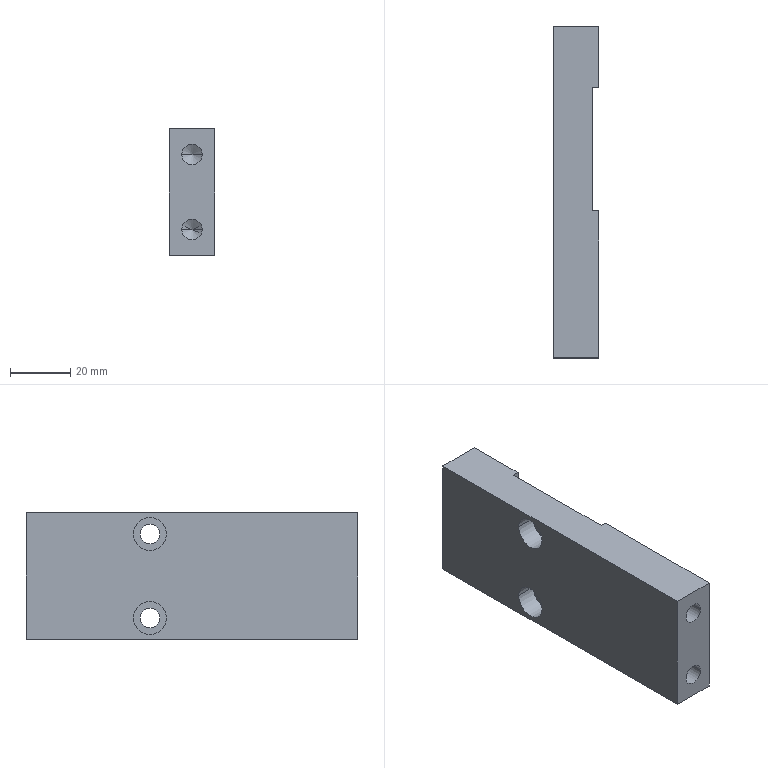Component | SolidWorks | CylinderBracket2-1 | 1 solid | 36 faces | box 15 x 110.5 x 42 mm | volume 62147 mm3 | cylinder 16 | plane 12 | cone 8 | commonest cylinder face diameters 3.3 x4 11 x4 6.6 x4 6.8 x4
build123d program:
from build123d import *

# Parameters (mm, degrees)
SKETCH2_W                                       = 15
SKETCH2_H                                       = 42
BOSS_EXTRUDE1_DEPTH                             = 138.5
M8_TAPPED_HOLE1_D                               = 6.8
M8_TAPPED_HOLE1_DEPTH                           = 25
M8_TAPPED_HOLE1_TIP                             = 2.043
SKETCH7_W                                       = 2
SKETCH7_H                                       = 41.1
CUT_EXTRUDE1_DEPTH                              = 42
M6_HEX_SOCKET_HEAD_CAP_SCREW_CBORE1_D           = 6.6
M6_HEX_SOCKET_HEAD_CAP_SCREW_CBORE1_CBORE_D     = 11
M6_HEX_SOCKET_HEAD_CAP_SCREW_CBORE1_CBORE_DEPTH = 6.8
SKETCH10_W                                      = 15
SKETCH10_H                                      = 28
CUT_EXTRUDE2_DEPTH                              = 53
M4_TAPPED_HOLE1_D                               = 3.3
M4_TAPPED_HOLE1_DEPTH                           = 25
M4_TAPPED_HOLE1_TIP                             = 0.9914


with BuildPart() as part:
    # Sketch2 → Boss-Extrude1 (new body)
    with BuildSketch(Plane.XY):
        with Locations((-3.66, -1.392)):
            Rectangle(SKETCH2_W, SKETCH2_H)
    extrude(amount=BOSS_EXTRUDE1_DEPTH)

    # M8 Tapped Hole1
    with Locations(Plane.XY.offset(138.5)):
        with Locations((-3.66, 11.108), (-3.66, -13.892)):
            Hole(M8_TAPPED_HOLE1_D / 2, depth=M8_TAPPED_HOLE1_DEPTH)
            with Locations((0, 0, -(M8_TAPPED_HOLE1_DEPTH + M8_TAPPED_HOLE1_TIP / 2))):  # 118° drill point
                Cone(0, M8_TAPPED_HOLE1_D / 2, M8_TAPPED_HOLE1_TIP, mode=Mode.SUBTRACT)

    # Sketch7 → Cut-Extrude1 (cut)
    with BuildSketch(Plane.XZ.offset(22.392)):
        with Locations((2.84, 69)):
            Rectangle(SKETCH7_W, SKETCH7_H)
    extrude(amount=-CUT_EXTRUDE1_DEPTH, mode=Mode.SUBTRACT)

    # M6 Hex Socket Head Cap Screw CBORE1 (through all)
    with Locations(Plane.ZY.offset(11.16)):
        with Locations((69.25, 12.608), (69.25, -15.392)):
            CounterBoreHole(M6_HEX_SOCKET_HEAD_CAP_SCREW_CBORE1_D / 2, M6_HEX_SOCKET_HEAD_CAP_SCREW_CBORE1_CBORE_D / 2, M6_HEX_SOCKET_HEAD_CAP_SCREW_CBORE1_CBORE_DEPTH)

    # Sketch10 → Cut-Extrude2 (cut)
    with BuildSketch(Plane.XZ.offset(22.392)):
        with Locations((-3.66, 14)):
            Rectangle(SKETCH10_W, SKETCH10_H)
    extrude(amount=-CUT_EXTRUDE2_DEPTH, mode=Mode.SUBTRACT)

    # M4 Tapped Hole1
    with Locations(Plane(origin=(0, 0, 28), x_dir=(-1, 0, 0), z_dir=(0, 0, -1))):
        with Locations((3.66, -18.392), (3.66, 15.608)):
            Hole(M4_TAPPED_HOLE1_D / 2, depth=M4_TAPPED_HOLE1_DEPTH)
            with Locations((0, 0, -(M4_TAPPED_HOLE1_DEPTH + M4_TAPPED_HOLE1_TIP / 2))):  # 118° drill point
                Cone(0, M4_TAPPED_HOLE1_D / 2, M4_TAPPED_HOLE1_TIP, mode=Mode.SUBTRACT)


solid = part.part

# Placed as in the assembly
solid = solid.moved(Location((-635.536, -9.151, 375.56), (90, 0, 0)))
STEP:
#1=CARTESIAN_POINT('',(-25.165,-2.447,13.997));
#2=VERTEX_POINT('',#1);
#3=CARTESIAN_POINT('',(-25.165,-2.447,14.127));
#4=VERTEX_POINT('',#3);
#5=CARTESIAN_POINT('',(-25.165,-2.447,14.062));
#6=DIRECTION('',(-0.,1.,-0.));
#7=DIRECTION('',(0.,0.,1.));
#8=AXIS2_PLACEMENT_3D('',#5,#6,#7);
#9=CIRCLE('',#8,0.06496);
#10=EDGE_CURVE('',#2,#4,#9,.T.);
#11=ORIENTED_EDGE('',*,*,#10,.F.);
#12=CARTESIAN_POINT('',(-25.165,-1.463,13.997));
#13=VERTEX_POINT('',#12);
#14=CARTESIAN_POINT('',(-25.165,-1.463,13.997));
#15=DIRECTION('',(-0.,1.,-0.));
#16=VECTOR('',#15,39.37);
#17=LINE('',#14,#16);
#18=EDGE_CURVE('',#2,#13,#17,.T.);
#19=ORIENTED_EDGE('',*,*,#18,.T.);
#20=CARTESIAN_POINT('',(-25.165,-1.463,14.127));
#21=VERTEX_POINT('',#20);
#22=CARTESIAN_POINT('',(-25.165,-1.463,14.062));
#23=DIRECTION('',(-0.,1.,-0.));
#24=DIRECTION('',(0.,0.,1.));
#25=AXIS2_PLACEMENT_3D('',#22,#23,#24);
#26=CIRCLE('',#25,0.06496);
#27=EDGE_CURVE('',#13,#21,#26,.T.);
#28=ORIENTED_EDGE('',*,*,#27,.T.);
#29=CARTESIAN_POINT('',(-25.165,-1.463,14.127));
#30=DIRECTION('',(-0.,1.,-0.));
#31=VECTOR('',#30,39.37);
#32=LINE('',#29,#31);
#33=EDGE_CURVE('',#4,#21,#32,.T.);
#34=ORIENTED_EDGE('',*,*,#33,.F.);
#35=EDGE_LOOP('',(#11,#19,#28,#34));
#36=FACE_OUTER_BOUND('',#35,.T.);
#37=CARTESIAN_POINT('',(-25.165,-1.463,14.062));
#38=DIRECTION('',(-0.,1.,-0.));
#39=DIRECTION('',(0.,0.,1.));
#40=AXIS2_PLACEMENT_3D('',#37,#38,#39);
#41=CYLINDRICAL_SURFACE('',#40,0.06496);
#42=ADVANCED_FACE('',(#36),#41,.F.);
#43=CARTESIAN_POINT('',(-25.165,-2.486,14.062));
#44=VERTEX_POINT('',#43);
#45=CARTESIAN_POINT('',(-25.165,-2.447,14.127));
#46=DIRECTION('',(-0.,0.515,0.8572));
#47=VECTOR('',#46,39.37);
#48=LINE('',#45,#47);
#49=EDGE_CURVE('',#44,#4,#48,.T.);
#50=ORIENTED_EDGE('',*,*,#49,.F.);
#51=CARTESIAN_POINT('',(-25.165,-2.447,13.997));
#52=DIRECTION('',(0.,0.515,-0.8572));
#53=VECTOR('',#52,39.37);
#54=LINE('',#51,#53);
#55=EDGE_CURVE('',#44,#2,#54,.T.);
#56=ORIENTED_EDGE('',*,*,#55,.T.);
#57=ORIENTED_EDGE('',*,*,#10,.T.);
#58=EDGE_LOOP('',(#50,#56,#57));
#59=FACE_OUTER_BOUND('',#58,.T.);
#60=CARTESIAN_POINT('',(-25.165,-2.447,14.062));
#61=DIRECTION('',(-0.,1.,-0.));
#62=DIRECTION('',(0.,0.,1.));
#63=AXIS2_PLACEMENT_3D('',#60,#61,#62);
#64=CONICAL_SURFACE('',#63,0.06496,1.03);
#65=ADVANCED_FACE('',(#59),#64,.F.);
#66=CARTESIAN_POINT('',(-25.165,-2.447,15.335));
#67=VERTEX_POINT('',#66);
#68=CARTESIAN_POINT('',(-25.165,-2.447,15.465));
#69=VERTEX_POINT('',#68);
#70=CARTESIAN_POINT('',(-25.165,-2.447,15.4));
#71=DIRECTION('',(-0.,1.,-0.));
#72=DIRECTION('',(0.,0.,1.));
#73=AXIS2_PLACEMENT_3D('',#70,#71,#72);
#74=CIRCLE('',#73,0.06496);
#75=EDGE_CURVE('',#67,#69,#74,.T.);
#76=ORIENTED_EDGE('',*,*,#75,.F.);
#77=CARTESIAN_POINT('',(-25.165,-1.463,15.335));
#78=VERTEX_POINT('',#77);
#79=CARTESIAN_POINT('',(-25.165,-1.463,15.335));
#80=DIRECTION('',(-0.,1.,-0.));
#81=VECTOR('',#80,39.37);
#82=LINE('',#79,#81);
#83=EDGE_CURVE('',#67,#78,#82,.T.);
#84=ORIENTED_EDGE('',*,*,#83,.T.);
#85=CARTESIAN_POINT('',(-25.165,-1.463,15.465));
#86=VERTEX_POINT('',#85);
#87=CARTESIAN_POINT('',(-25.165,-1.463,15.4));
#88=DIRECTION('',(-0.,1.,-0.));
#89=DIRECTION('',(0.,0.,1.));
#90=AXIS2_PLACEMENT_3D('',#87,#88,#89);
#91=CIRCLE('',#90,0.06496);
#92=EDGE_CURVE('',#78,#86,#91,.T.);
#93=ORIENTED_EDGE('',*,*,#92,.T.);
#94=CARTESIAN_POINT('',(-25.165,-1.463,15.465));
#95=DIRECTION('',(-0.,1.,-0.));
#96=VECTOR('',#95,39.37);
#97=LINE('',#94,#96);
#98=EDGE_CURVE('',#69,#86,#97,.T.);
#99=ORIENTED_EDGE('',*,*,#98,.F.);
#100=EDGE_LOOP('',(#76,#84,#93,#99));
#101=FACE_OUTER_BOUND('',#100,.T.);
#102=CARTESIAN_POINT('',(-25.165,-1.463,15.4));
#103=DIRECTION('',(-0.,1.,-0.));
#104=DIRECTION('',(0.,0.,1.));
#105=AXIS2_PLACEMENT_3D('',#102,#103,#104);
#106=CYLINDRICAL_SURFACE('',#105,0.06496);
#107=ADVANCED_FACE('',(#101),#106,.F.);
#108=CARTESIAN_POINT('',(-25.165,-2.486,15.4));
#109=VERTEX_POINT('',#108);
#110=CARTESIAN_POINT('',(-25.165,-2.447,15.465));
#111=DIRECTION('',(-0.,0.515,0.8572));
#112=VECTOR('',#111,39.37);
#113=LINE('',#110,#112);
#114=EDGE_CURVE('',#109,#69,#113,.T.);
#115=ORIENTED_EDGE('',*,*,#114,.F.);
#116=CARTESIAN_POINT('',(-25.165,-2.447,15.335));
#117=DIRECTION('',(0.,0.515,-0.8572));
#118=VECTOR('',#117,39.37);
#119=LINE('',#116,#118);
#120=EDGE_CURVE('',#109,#67,#119,.T.);
#121=ORIENTED_EDGE('',*,*,#120,.T.);
#122=ORIENTED_EDGE('',*,*,#75,.T.);
#123=EDGE_LOOP('',(#115,#121,#122));
#124=FACE_OUTER_BOUND('',#123,.T.);
#125=CARTESIAN_POINT('',(-25.165,-2.447,15.4));
#126=DIRECTION('',(-0.,1.,-0.));
#127=DIRECTION('',(0.,0.,1.));
#128=AXIS2_PLACEMENT_3D('',#125,#126,#127);
#129=CONICAL_SURFACE('',#128,0.06496,1.03);
#130=ADVANCED_FACE('',(#124),#129,.F.);
#131=CARTESIAN_POINT('',(-25.193,-2.87,14.18));
#132=VERTEX_POINT('',#131);
#133=CARTESIAN_POINT('',(-25.193,-3.303,14.18));
#134=VERTEX_POINT('',#133);
#135=CARTESIAN_POINT('',(-25.193,-3.087,14.18));
#136=DIRECTION('',(-1.,-0.,-0.));
#137=DIRECTION('',(0.,-1.,0.));
#138=AXIS2_PLACEMENT_3D('',#135,#136,#137);
#139=CIRCLE('',#138,0.2165);
#140=EDGE_CURVE('',#132,#134,#139,.T.);
#141=ORIENTED_EDGE('',*,*,#140,.F.);
#142=CARTESIAN_POINT('',(-25.46,-2.87,14.18));
#143=VERTEX_POINT('',#142);
#144=CARTESIAN_POINT('',(-25.46,-2.87,14.18));
#145=DIRECTION('',(-1.,-0.,-0.));
#146=VECTOR('',#145,39.37);
#147=LINE('',#144,#146);
#148=EDGE_CURVE('',#132,#143,#147,.T.);
#149=ORIENTED_EDGE('',*,*,#148,.T.);
#150=CARTESIAN_POINT('',(-25.46,-3.303,14.18));
#151=VERTEX_POINT('',#150);
#152=CARTESIAN_POINT('',(-25.46,-3.087,14.18));
#153=DIRECTION('',(-1.,-0.,-0.));
#154=DIRECTION('',(0.,-1.,0.));
#155=AXIS2_PLACEMENT_3D('',#152,#153,#154);
#156=CIRCLE('',#155,0.2165);
#157=EDGE_CURVE('',#143,#151,#156,.T.);
#158=ORIENTED_EDGE('',*,*,#157,.T.);
#159=CARTESIAN_POINT('',(-25.46,-3.303,14.18));
#160=DIRECTION('',(-1.,-0.,-0.));
#161=VECTOR('',#160,39.37);
#162=LINE('',#159,#161);
#163=EDGE_CURVE('',#134,#151,#162,.T.);
#164=ORIENTED_EDGE('',*,*,#163,.F.);
#165=EDGE_LOOP('',(#141,#149,#158,#164));
#166=FACE_OUTER_BOUND('',#165,.T.);
#167=CARTESIAN_POINT('',(-25.46,-3.087,14.18));
#168=DIRECTION('',(-1.,-0.,-0.));
#169=DIRECTION('',(0.,-1.,0.));
#170=AXIS2_PLACEMENT_3D('',#167,#168,#169);
#171=CYLINDRICAL_SURFACE('',#170,0.2165);
#172=ADVANCED_FACE('',(#166),#171,.F.);
#173=CARTESIAN_POINT('',(-24.949,-2.957,14.18));
#174=VERTEX_POINT('',#173);
#175=CARTESIAN_POINT('',(-24.949,-3.217,14.18));
#176=VERTEX_POINT('',#175);
#177=CARTESIAN_POINT('',(-24.949,-3.087,14.18));
#178=DIRECTION('',(-1.,-0.,-0.));
#179=DIRECTION('',(0.,0.,-1.));
#180=AXIS2_PLACEMENT_3D('',#177,#178,#179);
#181=CIRCLE('',#180,0.1299);
#182=EDGE_CURVE('',#174,#176,#181,.T.);
#183=ORIENTED_EDGE('',*,*,#182,.F.);
#184=CARTESIAN_POINT('',(-25.193,-2.957,14.18));
#185=VERTEX_POINT('',#184);
#186=CARTESIAN_POINT('',(-25.46,-2.957,14.18));
#187=DIRECTION('',(-1.,-0.,-0.));
#188=VECTOR('',#187,39.37);
#189=LINE('',#186,#188);
#190=EDGE_CURVE('',#174,#185,#189,.T.);
#191=ORIENTED_EDGE('',*,*,#190,.T.);
#192=CARTESIAN_POINT('',(-25.193,-3.217,14.18));
#193=VERTEX_POINT('',#192);
#194=CARTESIAN_POINT('',(-25.193,-3.087,14.18));
#195=DIRECTION('',(-1.,-0.,-0.));
#196=DIRECTION('',(0.,-1.,0.));
#197=AXIS2_PLACEMENT_3D('',#194,#195,#196);
#198=CIRCLE('',#197,0.1299);
#199=EDGE_CURVE('',#185,#193,#198,.T.);
#200=ORIENTED_EDGE('',*,*,#199,.T.);
#201=CARTESIAN_POINT('',(-25.46,-3.217,14.18));
#202=DIRECTION('',(-1.,-0.,-0.));
#203=VECTOR('',#202,39.37);
#204=LINE('',#201,#203);
#205=EDGE_CURVE('',#176,#193,#204,.T.);
#206=ORIENTED_EDGE('',*,*,#205,.F.);
#207=EDGE_LOOP('',(#183,#191,#200,#206));
#208=FACE_OUTER_BOUND('',#207,.T.);
#209=CARTESIAN_POINT('',(-25.46,-3.087,14.18));
#210=DIRECTION('',(-1.,-0.,-0.));
#211=DIRECTION('',(0.,-1.,0.));
#212=AXIS2_PLACEMENT_3D('',#209,#210,#211);
#213=CYLINDRICAL_SURFACE('',#212,0.1299);
#214=ADVANCED_FACE('',(#208),#213,.F.);
#215=CARTESIAN_POINT('',(-25.193,-2.87,15.282));
#216=VERTEX_POINT('',#215);
#217=CARTESIAN_POINT('',(-25.193,-3.303,15.282));
#218=VERTEX_POINT('',#217);
#219=CARTESIAN_POINT('',(-25.193,-3.087,15.282));
#220=DIRECTION('',(-1.,-0.,-0.));
#221=DIRECTION('',(0.,-1.,0.));
#222=AXIS2_PLACEMENT_3D('',#219,#220,#221);
#223=CIRCLE('',#222,0.2165);
#224=EDGE_CURVE('',#216,#218,#223,.T.);
#225=ORIENTED_EDGE('',*,*,#224,.F.);
#226=CARTESIAN_POINT('',(-25.46,-2.87,15.282));
#227=VERTEX_POINT('',#226);
#228=CARTESIAN_POINT('',(-25.46,-2.87,15.282));
#229=DIRECTION('',(-1.,-0.,-0.));
#230=VECTOR('',#229,39.37);
#231=LINE('',#228,#230);
#232=EDGE_CURVE('',#216,#227,#231,.T.);
#233=ORIENTED_EDGE('',*,*,#232,.T.);
#234=CARTESIAN_POINT('',(-25.46,-3.303,15.282));
#235=VERTEX_POINT('',#234);
#236=CARTESIAN_POINT('',(-25.46,-3.087,15.282));
#237=DIRECTION('',(-1.,-0.,-0.));
#238=DIRECTION('',(0.,-1.,0.));
#239=AXIS2_PLACEMENT_3D('',#236,#237,#238);
#240=CIRCLE('',#239,0.2165);
#241=EDGE_CURVE('',#227,#235,#240,.T.);
#242=ORIENTED_EDGE('',*,*,#241,.T.);
#243=CARTESIAN_POINT('',(-25.46,-3.303,15.282));
#244=DIRECTION('',(-1.,-0.,-0.));
#245=VECTOR('',#244,39.37);
#246=LINE('',#243,#245);
#247=EDGE_CURVE('',#218,#235,#246,.T.);
#248=ORIENTED_EDGE('',*,*,#247,.F.);
#249=EDGE_LOOP('',(#225,#233,#242,#248));
#250=FACE_OUTER_BOUND('',#249,.T.);
#251=CARTESIAN_POINT('',(-25.46,-3.087,15.282));
#252=DIRECTION('',(-1.,-0.,-0.));
#253=DIRECTION('',(0.,-1.,0.));
#254=AXIS2_PLACEMENT_3D('',#251,#252,#253);
#255=CYLINDRICAL_SURFACE('',#254,0.2165);
#256=ADVANCED_FACE('',(#250),#255,.F.);
#257=CARTESIAN_POINT('',(-24.949,-2.957,15.282));
#258=VERTEX_POINT('',#257);
#259=CARTESIAN_POINT('',(-24.949,-3.217,15.282));
#260=VERTEX_POINT('',#259);
#261=CARTESIAN_POINT('',(-24.949,-3.087,15.282));
#262=DIRECTION('',(-1.,-0.,-0.));
#263=DIRECTION('',(0.,0.,-1.));
#264=AXIS2_PLACEMENT_3D('',#261,#262,#263);
#265=CIRCLE('',#264,0.1299);
#266=EDGE_CURVE('',#258,#260,#265,.T.);
#267=ORIENTED_EDGE('',*,*,#266,.F.);
#268=CARTESIAN_POINT('',(-25.193,-2.957,15.282));
#269=VERTEX_POINT('',#268);
#270=CARTESIAN_POINT('',(-25.46,-2.957,15.282));
#271=DIRECTION('',(-1.,-0.,-0.));
#272=VECTOR('',#271,39.37);
#273=LINE('',#270,#272);
#274=EDGE_CURVE('',#258,#269,#273,.T.);
#275=ORIENTED_EDGE('',*,*,#274,.T.);
#276=CARTESIAN_POINT('',(-25.193,-3.217,15.282));
#277=VERTEX_POINT('',#276);
#278=CARTESIAN_POINT('',(-25.193,-3.087,15.282));
#279=DIRECTION('',(-1.,-0.,-0.));
#280=DIRECTION('',(0.,-1.,0.));
#281=AXIS2_PLACEMENT_3D('',#278,#279,#280);
#282=CIRCLE('',#281,0.1299);
#283=EDGE_CURVE('',#269,#277,#282,.T.);
#284=ORIENTED_EDGE('',*,*,#283,.T.);
#285=CARTESIAN_POINT('',(-25.46,-3.217,15.282));
#286=DIRECTION('',(-1.,-0.,-0.));
#287=VECTOR('',#286,39.37);
#288=LINE('',#285,#287);
#289=EDGE_CURVE('',#260,#277,#288,.T.);
#290=ORIENTED_EDGE('',*,*,#289,.F.);
#291=EDGE_LOOP('',(#267,#275,#284,#290));
#292=FACE_OUTER_BOUND('',#291,.T.);
#293=CARTESIAN_POINT('',(-25.46,-3.087,15.282));
#294=DIRECTION('',(-1.,-0.,-0.));
#295=DIRECTION('',(0.,-1.,0.));
#296=AXIS2_PLACEMENT_3D('',#293,#294,#295);
#297=CYLINDRICAL_SURFACE('',#296,0.1299);
#298=ADVANCED_FACE('',(#292),#297,.F.);
#299=CARTESIAN_POINT('',(-25.299,-4.829,14.239));
#300=VERTEX_POINT('',#299);
#301=CARTESIAN_POINT('',(-25.031,-4.829,14.239));
#302=VERTEX_POINT('',#301);
#303=CARTESIAN_POINT('',(-25.165,-4.829,14.239));
#304=DIRECTION('',(0.,-1.,0.));
#305=DIRECTION('',(1.,0.,0.));
#306=AXIS2_PLACEMENT_3D('',#303,#304,#305);
#307=CIRCLE('',#306,0.1339);
#308=EDGE_CURVE('',#300,#302,#307,.T.);
#309=ORIENTED_EDGE('',*,*,#308,.F.);
#310=CARTESIAN_POINT('',(-25.299,-5.813,14.239));
#311=VERTEX_POINT('',#310);
#312=CARTESIAN_POINT('',(-25.299,-5.813,14.239));
#313=DIRECTION('',(0.,-1.,0.));
#314=VECTOR('',#313,39.37);
#315=LINE('',#312,#314);
#316=EDGE_CURVE('',#300,#311,#315,.T.);
#317=ORIENTED_EDGE('',*,*,#316,.T.);
#318=CARTESIAN_POINT('',(-25.031,-5.813,14.239));
#319=VERTEX_POINT('',#318);
#320=CARTESIAN_POINT('',(-25.165,-5.813,14.239));
#321=DIRECTION('',(0.,-1.,0.));
#322=DIRECTION('',(1.,0.,0.));
#323=AXIS2_PLACEMENT_3D('',#320,#321,#322);
#324=CIRCLE('',#323,0.1339);
#325=EDGE_CURVE('',#311,#319,#324,.T.);
#326=ORIENTED_EDGE('',*,*,#325,.T.);
#327=CARTESIAN_POINT('',(-25.031,-5.813,14.239));
#328=DIRECTION('',(0.,-1.,0.));
#329=VECTOR('',#328,39.37);
#330=LINE('',#327,#329);
#331=EDGE_CURVE('',#302,#319,#330,.T.);
#332=ORIENTED_EDGE('',*,*,#331,.F.);
#333=EDGE_LOOP('',(#309,#317,#326,#332));
#334=FACE_OUTER_BOUND('',#333,.T.);
#335=CARTESIAN_POINT('',(-25.165,-5.813,14.239));
#336=DIRECTION('',(0.,-1.,0.));
#337=DIRECTION('',(1.,0.,0.));
#338=AXIS2_PLACEMENT_3D('',#335,#336,#337);
#339=CYLINDRICAL_SURFACE('',#338,0.1339);
#340=ADVANCED_FACE('',(#334),#339,.F.);
#341=CARTESIAN_POINT('',(-25.165,-4.748,14.239));
#342=VERTEX_POINT('',#341);
#343=CARTESIAN_POINT('',(-25.031,-4.829,14.239));
#344=DIRECTION('',(0.8572,-0.515,0.));
#345=VECTOR('',#344,39.37);
#346=LINE('',#343,#345);
#347=EDGE_CURVE('',#342,#302,#346,.T.);
#348=ORIENTED_EDGE('',*,*,#347,.F.);
#349=CARTESIAN_POINT('',(-25.299,-4.829,14.239));
#350=DIRECTION('',(-0.8572,-0.515,0.));
#351=VECTOR('',#350,39.37);
#352=LINE('',#349,#351);
#353=EDGE_CURVE('',#342,#300,#352,.T.);
#354=ORIENTED_EDGE('',*,*,#353,.T.);
#355=ORIENTED_EDGE('',*,*,#308,.T.);
#356=EDGE_LOOP('',(#348,#354,#355));
#357=FACE_OUTER_BOUND('',#356,.T.);
#358=CARTESIAN_POINT('',(-25.165,-4.829,14.239));
#359=DIRECTION('',(0.,-1.,0.));
#360=DIRECTION('',(1.,0.,0.));
#361=AXIS2_PLACEMENT_3D('',#358,#359,#360);
#362=CONICAL_SURFACE('',#361,0.1339,1.03);
#363=ADVANCED_FACE('',(#357),#362,.F.);
#364=CARTESIAN_POINT('',(-25.299,-4.829,15.223));
#365=VERTEX_POINT('',#364);
#366=CARTESIAN_POINT('',(-25.031,-4.829,15.223));
#367=VERTEX_POINT('',#366);
#368=CARTESIAN_POINT('',(-25.165,-4.829,15.223));
#369=DIRECTION('',(0.,-1.,0.));
#370=DIRECTION('',(1.,0.,0.));
#371=AXIS2_PLACEMENT_3D('',#368,#369,#370);
#372=CIRCLE('',#371,0.1339);
#373=EDGE_CURVE('',#365,#367,#372,.T.);
#374=ORIENTED_EDGE('',*,*,#373,.F.);
#375=CARTESIAN_POINT('',(-25.299,-5.813,15.223));
#376=VERTEX_POINT('',#375);
#377=CARTESIAN_POINT('',(-25.299,-5.813,15.223));
#378=DIRECTION('',(0.,-1.,0.));
#379=VECTOR('',#378,39.37);
#380=LINE('',#377,#379);
#381=EDGE_CURVE('',#365,#376,#380,.T.);
#382=ORIENTED_EDGE('',*,*,#381,.T.);
#383=CARTESIAN_POINT('',(-25.031,-5.813,15.223));
#384=VERTEX_POINT('',#383);
#385=CARTESIAN_POINT('',(-25.165,-5.813,15.223));
#386=DIRECTION('',(0.,-1.,0.));
#387=DIRECTION('',(1.,0.,0.));
#388=AXIS2_PLACEMENT_3D('',#385,#386,#387);
#389=CIRCLE('',#388,0.1339);
#390=EDGE_CURVE('',#376,#384,#389,.T.);
#391=ORIENTED_EDGE('',*,*,#390,.T.);
#392=CARTESIAN_POINT('',(-25.031,-5.813,15.223));
#393=DIRECTION('',(0.,-1.,0.));
#394=VECTOR('',#393,39.37);
#395=LINE('',#392,#394);
#396=EDGE_CURVE('',#367,#384,#395,.T.);
#397=ORIENTED_EDGE('',*,*,#396,.F.);
#398=EDGE_LOOP('',(#374,#382,#391,#397));
#399=FACE_OUTER_BOUND('',#398,.T.);
#400=CARTESIAN_POINT('',(-25.165,-5.813,15.223));
#401=DIRECTION('',(0.,-1.,0.));
#402=DIRECTION('',(1.,0.,0.));
#403=AXIS2_PLACEMENT_3D('',#400,#401,#402);
#404=CYLINDRICAL_SURFACE('',#403,0.1339);
#405=ADVANCED_FACE('',(#399),#404,.F.);
#406=CARTESIAN_POINT('',(-25.165,-4.748,15.223));
#407=VERTEX_POINT('',#406);
#408=CARTESIAN_POINT('',(-25.031,-4.829,15.223));
#409=DIRECTION('',(0.8572,-0.515,0.));
#410=VECTOR('',#409,39.37);
#411=LINE('',#408,#410);
#412=EDGE_CURVE('',#407,#367,#411,.T.);
#413=ORIENTED_EDGE('',*,*,#412,.F.);
#414=CARTESIAN_POINT('',(-25.299,-4.829,15.223));
#415=DIRECTION('',(-0.8572,-0.515,0.));
#416=VECTOR('',#415,39.37);
#417=LINE('',#414,#416);
#418=EDGE_CURVE('',#407,#365,#417,.T.);
#419=ORIENTED_EDGE('',*,*,#418,.T.);
#420=ORIENTED_EDGE('',*,*,#373,.T.);
#421=EDGE_LOOP('',(#413,#419,#420));
#422=FACE_OUTER_BOUND('',#421,.T.);
#423=CARTESIAN_POINT('',(-25.165,-4.829,15.223));
#424=DIRECTION('',(0.,-1.,0.));
#425=DIRECTION('',(1.,0.,0.));
#426=AXIS2_PLACEMENT_3D('',#423,#424,#425);
#427=CONICAL_SURFACE('',#426,0.1339,1.03);
#428=ADVANCED_FACE('',(#422),#427,.F.);
#429=CARTESIAN_POINT('',(-24.87,-2.268,13.904));
#430=VERTEX_POINT('',#429);
#431=CARTESIAN_POINT('',(-24.87,-1.463,13.904));
#432=VERTEX_POINT('',#431);
#433=CARTESIAN_POINT('',(-24.87,-5.813,13.904));
#434=DIRECTION('',(-0.,1.,-0.));
#435=VECTOR('',#434,39.37);
#436=LINE('',#433,#435);
#437=EDGE_CURVE('',#430,#432,#436,.T.);
#438=ORIENTED_EDGE('',*,*,#437,.T.);
#439=CARTESIAN_POINT('',(-24.87,-1.463,15.558));
#440=VERTEX_POINT('',#439);
#441=CARTESIAN_POINT('',(-24.87,-1.463,15.991));
#442=DIRECTION('',(0.,-0.,-1.));
#443=VECTOR('',#442,39.37);
#444=LINE('',#441,#443);
#445=EDGE_CURVE('',#440,#432,#444,.T.);
#446=ORIENTED_EDGE('',*,*,#445,.F.);
#447=CARTESIAN_POINT('',(-24.87,-2.268,15.558));
#448=VERTEX_POINT('',#447);
#449=CARTESIAN_POINT('',(-24.87,-5.813,15.558));
#450=DIRECTION('',(-0.,1.,-0.));
#451=VECTOR('',#450,39.37);
#452=LINE('',#449,#451);
#453=EDGE_CURVE('',#448,#440,#452,.T.);
#454=ORIENTED_EDGE('',*,*,#453,.F.);
#455=CARTESIAN_POINT('',(-24.87,-2.268,15.558));
#456=DIRECTION('',(0.,-0.,-1.));
#457=VECTOR('',#456,39.37);
#458=LINE('',#455,#457);
#459=EDGE_CURVE('',#448,#430,#458,.T.);
#460=ORIENTED_EDGE('',*,*,#459,.T.);
#461=EDGE_LOOP('',(#438,#446,#454,#460));
#462=FACE_OUTER_BOUND('',#461,.T.);
#463=CARTESIAN_POINT('',(-24.87,-5.813,15.558));
#464=DIRECTION('',(-1.,-0.,-0.));
#465=DIRECTION('',(0.,-0.,-1.));
#466=AXIS2_PLACEMENT_3D('',#463,#464,#465);
#467=PLANE('',#466);
#468=ADVANCED_FACE('',(#462),#467,.F.);
#469=CARTESIAN_POINT('',(-25.46,-3.087,14.18));
#470=DIRECTION('',(-1.,-0.,-0.));
#471=DIRECTION('',(0.,-1.,0.));
#472=AXIS2_PLACEMENT_3D('',#469,#470,#471);
#473=CIRCLE('',#472,0.2165);
#474=EDGE_CURVE('',#151,#143,#473,.T.);
#475=ORIENTED_EDGE('',*,*,#474,.F.);
#476=ORIENTED_EDGE('',*,*,#157,.F.);
#477=EDGE_LOOP('',(#475,#476));
#478=FACE_BOUND('',#477,.T.);
#479=CARTESIAN_POINT('',(-25.46,-3.087,15.282));
#480=DIRECTION('',(-1.,-0.,-0.));
#481=DIRECTION('',(0.,-1.,0.));
#482=AXIS2_PLACEMENT_3D('',#479,#480,#481);
#483=CIRCLE('',#482,0.2165);
#484=EDGE_CURVE('',#235,#227,#483,.T.);
#485=ORIENTED_EDGE('',*,*,#484,.F.);
#486=ORIENTED_EDGE('',*,*,#241,.F.);
#487=EDGE_LOOP('',(#485,#486));
#488=FACE_BOUND('',#487,.T.);
#489=CARTESIAN_POINT('',(-25.46,-5.813,15.558));
#490=VERTEX_POINT('',#489);
#491=CARTESIAN_POINT('',(-25.46,-1.463,15.558));
#492=VERTEX_POINT('',#491);
#493=CARTESIAN_POINT('',(-25.46,-5.813,15.558));
#494=DIRECTION('',(-0.,1.,-0.));
#495=VECTOR('',#494,39.37);
#496=LINE('',#493,#495);
#497=EDGE_CURVE('',#490,#492,#496,.T.);
#498=ORIENTED_EDGE('',*,*,#497,.T.);
#499=CARTESIAN_POINT('',(-25.46,-1.463,13.904));
#500=VERTEX_POINT('',#499);
#501=CARTESIAN_POINT('',(-25.46,-1.463,15.991));
#502=DIRECTION('',(0.,-0.,-1.));
#503=VECTOR('',#502,39.37);
#504=LINE('',#501,#503);
#505=EDGE_CURVE('',#492,#500,#504,.T.);
#506=ORIENTED_EDGE('',*,*,#505,.T.);
#507=CARTESIAN_POINT('',(-25.46,-5.813,13.904));
#508=VERTEX_POINT('',#507);
#509=CARTESIAN_POINT('',(-25.46,-5.813,13.904));
#510=DIRECTION('',(-0.,1.,-0.));
#511=VECTOR('',#510,39.37);
#512=LINE('',#509,#511);
#513=EDGE_CURVE('',#508,#500,#512,.T.);
#514=ORIENTED_EDGE('',*,*,#513,.F.);
#515=CARTESIAN_POINT('',(-25.46,-5.813,15.558));
#516=DIRECTION('',(0.,-0.,-1.));
#517=VECTOR('',#516,39.37);
#518=LINE('',#515,#517);
#519=EDGE_CURVE('',#490,#508,#518,.T.);
#520=ORIENTED_EDGE('',*,*,#519,.F.);
#521=EDGE_LOOP('',(#498,#506,#514,#520));
#522=FACE_OUTER_BOUND('',#521,.T.);
#523=CARTESIAN_POINT('',(-25.46,-5.813,15.558));
#524=DIRECTION('',(1.,0.,0.));
#525=DIRECTION('',(-0.,0.,1.));
#526=AXIS2_PLACEMENT_3D('',#523,#524,#525);
#527=PLANE('',#526);
#528=ADVANCED_FACE('',(#478,#488,#522),#527,.F.);
#529=ORIENTED_EDGE('',*,*,#513,.T.);
#530=CARTESIAN_POINT('',(-24.87,-1.463,13.904));
#531=DIRECTION('',(-1.,0.,-0.));
#532=VECTOR('',#531,39.37);
#533=LINE('',#530,#532);
#534=EDGE_CURVE('',#432,#500,#533,.T.);
#535=ORIENTED_EDGE('',*,*,#534,.F.);
#536=ORIENTED_EDGE('',*,*,#437,.F.);
#537=CARTESIAN_POINT('',(-24.949,-2.268,13.904));
#538=VERTEX_POINT('',#537);
#539=CARTESIAN_POINT('',(-24.87,-2.268,13.904));
#540=DIRECTION('',(1.,0.,0.));
#541=VECTOR('',#540,39.37);
#542=LINE('',#539,#541);
#543=EDGE_CURVE('',#538,#430,#542,.T.);
#544=ORIENTED_EDGE('',*,*,#543,.F.);
#545=CARTESIAN_POINT('',(-24.949,-3.886,13.904));
#546=VERTEX_POINT('',#545);
#547=CARTESIAN_POINT('',(-24.949,-2.268,13.904));
#548=DIRECTION('',(-0.,1.,-0.));
#549=VECTOR('',#548,39.37);
#550=LINE('',#547,#549);
#551=EDGE_CURVE('',#546,#538,#550,.T.);
#552=ORIENTED_EDGE('',*,*,#551,.F.);
#553=CARTESIAN_POINT('',(-24.87,-3.886,13.904));
#554=VERTEX_POINT('',#553);
#555=CARTESIAN_POINT('',(-24.87,-3.886,13.904));
#556=DIRECTION('',(-1.,-0.,-0.));
#557=VECTOR('',#556,39.37);
#558=LINE('',#555,#557);
#559=EDGE_CURVE('',#554,#546,#558,.T.);
#560=ORIENTED_EDGE('',*,*,#559,.F.);
#561=CARTESIAN_POINT('',(-24.87,-5.813,13.904));
#562=VERTEX_POINT('',#561);
#563=CARTESIAN_POINT('',(-24.87,-5.813,13.904));
#564=DIRECTION('',(-0.,1.,-0.));
#565=VECTOR('',#564,39.37);
#566=LINE('',#563,#565);
#567=EDGE_CURVE('',#562,#554,#566,.T.);
#568=ORIENTED_EDGE('',*,*,#567,.F.);
#569=CARTESIAN_POINT('',(-25.46,-5.813,13.904));
#570=DIRECTION('',(1.,0.,0.));
#571=VECTOR('',#570,39.37);
#572=LINE('',#569,#571);
#573=EDGE_CURVE('',#508,#562,#572,.T.);
#574=ORIENTED_EDGE('',*,*,#573,.F.);
#575=EDGE_LOOP('',(#529,#535,#536,#544,#552,#560,#568,#574));
#576=FACE_OUTER_BOUND('',#575,.T.);
#577=CARTESIAN_POINT('',(-25.46,-5.813,13.904));
#578=DIRECTION('',(-0.,0.,1.));
#579=DIRECTION('',(-1.,-0.,-0.));
#580=AXIS2_PLACEMENT_3D('',#577,#578,#579);
#581=PLANE('',#580);
#582=ADVANCED_FACE('',(#576),#581,.F.);
#583=ORIENTED_EDGE('',*,*,#567,.T.);
#584=CARTESIAN_POINT('',(-24.87,-3.886,15.558));
#585=VERTEX_POINT('',#584);
#586=CARTESIAN_POINT('',(-24.87,-3.886,15.558));
#587=DIRECTION('',(0.,-0.,-1.));
#588=VECTOR('',#587,39.37);
#589=LINE('',#586,#588);
#590=EDGE_CURVE('',#585,#554,#589,.T.);
#591=ORIENTED_EDGE('',*,*,#590,.F.);
#592=CARTESIAN_POINT('',(-24.87,-5.813,15.558));
#593=VERTEX_POINT('',#592);
#594=CARTESIAN_POINT('',(-24.87,-5.813,15.558));
#595=DIRECTION('',(-0.,1.,-0.));
#596=VECTOR('',#595,39.37);
#597=LINE('',#594,#596);
#598=EDGE_CURVE('',#593,#585,#597,.T.);
#599=ORIENTED_EDGE('',*,*,#598,.F.);
#600=CARTESIAN_POINT('',(-24.87,-5.813,15.558));
#601=DIRECTION('',(-0.,0.,1.));
#602=VECTOR('',#601,39.37);
#603=LINE('',#600,#602);
#604=EDGE_CURVE('',#562,#593,#603,.T.);
#605=ORIENTED_EDGE('',*,*,#604,.F.);
#606=EDGE_LOOP('',(#583,#591,#599,#605));
#607=FACE_OUTER_BOUND('',#606,.T.);
#608=CARTESIAN_POINT('',(-24.87,-5.813,15.558));
#609=DIRECTION('',(-1.,-0.,-0.));
#610=DIRECTION('',(0.,-0.,-1.));
#611=AXIS2_PLACEMENT_3D('',#608,#609,#610);
#612=PLANE('',#611);
#613=ADVANCED_FACE('',(#607),#612,.F.);
#614=ORIENTED_EDGE('',*,*,#453,.T.);
#615=CARTESIAN_POINT('',(-25.46,-1.463,15.558));
#616=DIRECTION('',(-1.,0.,-0.));
#617=VECTOR('',#616,39.37);
#618=LINE('',#615,#617);
#619=EDGE_CURVE('',#440,#492,#618,.T.);
#620=ORIENTED_EDGE('',*,*,#619,.T.);
#621=ORIENTED_EDGE('',*,*,#497,.F.);
#622=CARTESIAN_POINT('',(-25.46,-5.813,15.558));
#623=DIRECTION('',(-1.,-0.,-0.));
#624=VECTOR('',#623,39.37);
#625=LINE('',#622,#624);
#626=EDGE_CURVE('',#593,#490,#625,.T.);
#627=ORIENTED_EDGE('',*,*,#626,.F.);
#628=ORIENTED_EDGE('',*,*,#598,.T.);
#629=CARTESIAN_POINT('',(-24.949,-3.886,15.558));
#630=VERTEX_POINT('',#629);
#631=CARTESIAN_POINT('',(-24.87,-3.886,15.558));
#632=DIRECTION('',(-1.,-0.,-0.));
#633=VECTOR('',#632,39.37);
#634=LINE('',#631,#633);
#635=EDGE_CURVE('',#585,#630,#634,.T.);
#636=ORIENTED_EDGE('',*,*,#635,.T.);
#637=CARTESIAN_POINT('',(-24.949,-2.268,15.558));
#638=VERTEX_POINT('',#637);
#639=CARTESIAN_POINT('',(-24.949,-2.268,15.558));
#640=DIRECTION('',(-0.,1.,-0.));
#641=VECTOR('',#640,39.37);
#642=LINE('',#639,#641);
#643=EDGE_CURVE('',#630,#638,#642,.T.);
#644=ORIENTED_EDGE('',*,*,#643,.T.);
#645=CARTESIAN_POINT('',(-24.87,-2.268,15.558));
#646=DIRECTION('',(1.,0.,0.));
#647=VECTOR('',#646,39.37);
#648=LINE('',#645,#647);
#649=EDGE_CURVE('',#638,#448,#648,.T.);
#650=ORIENTED_EDGE('',*,*,#649,.T.);
#651=EDGE_LOOP('',(#614,#620,#621,#627,#628,#636,#644,#650));
#652=FACE_OUTER_BOUND('',#651,.T.);
#653=CARTESIAN_POINT('',(-25.46,-5.813,15.558));
#654=DIRECTION('',(0.,-0.,-1.));
#655=DIRECTION('',(1.,0.,0.));
#656=AXIS2_PLACEMENT_3D('',#653,#654,#655);
#657=PLANE('',#656);
#658=ADVANCED_FACE('',(#652),#657,.F.);
#659=CARTESIAN_POINT('',(-25.165,-5.813,14.239));
#660=DIRECTION('',(0.,-1.,0.));
#661=DIRECTION('',(1.,0.,0.));
#662=AXIS2_PLACEMENT_3D('',#659,#660,#661);
#663=CIRCLE('',#662,0.1339);
#664=EDGE_CURVE('',#319,#311,#663,.T.);
#665=ORIENTED_EDGE('',*,*,#664,.F.);
#666=ORIENTED_EDGE('',*,*,#325,.F.);
#667=EDGE_LOOP('',(#665,#666));
#668=FACE_BOUND('',#667,.T.);
#669=CARTESIAN_POINT('',(-25.165,-5.813,15.223));
#670=DIRECTION('',(0.,-1.,0.));
#671=DIRECTION('',(1.,0.,0.));
#672=AXIS2_PLACEMENT_3D('',#669,#670,#671);
#673=CIRCLE('',#672,0.1339);
#674=EDGE_CURVE('',#384,#376,#673,.T.);
#675=ORIENTED_EDGE('',*,*,#674,.F.);
#676=ORIENTED_EDGE('',*,*,#390,.F.);
#677=EDGE_LOOP('',(#675,#676));
#678=FACE_BOUND('',#677,.T.);
#679=ORIENTED_EDGE('',*,*,#519,.T.);
#680=ORIENTED_EDGE('',*,*,#573,.T.);
#681=ORIENTED_EDGE('',*,*,#604,.T.);
#682=ORIENTED_EDGE('',*,*,#626,.T.);
#683=EDGE_LOOP('',(#679,#680,#681,#682));
#684=FACE_OUTER_BOUND('',#683,.T.);
#685=CARTESIAN_POINT('',(-25.021,-5.813,14.786));
#686=DIRECTION('',(0.,-1.,0.));
#687=DIRECTION('',(1.,0.,0.));
#688=AXIS2_PLACEMENT_3D('',#685,#686,#687);
#689=PLANE('',#688);
#690=ADVANCED_FACE('',(#668,#678,#684),#689,.T.);
#691=ORIENTED_EDGE('',*,*,#418,.F.);
#692=ORIENTED_EDGE('',*,*,#412,.T.);
#693=CARTESIAN_POINT('',(-25.165,-4.829,15.223));
#694=DIRECTION('',(0.,-1.,0.));
#695=DIRECTION('',(1.,0.,0.));
#696=AXIS2_PLACEMENT_3D('',#693,#694,#695);
#697=CIRCLE('',#696,0.1339);
#698=EDGE_CURVE('',#367,#365,#697,.T.);
#699=ORIENTED_EDGE('',*,*,#698,.T.);
#700=EDGE_LOOP('',(#691,#692,#699));
#701=FACE_OUTER_BOUND('',#700,.T.);
#702=CARTESIAN_POINT('',(-25.165,-4.829,15.223));
#703=DIRECTION('',(0.,-1.,0.));
#704=DIRECTION('',(1.,0.,0.));
#705=AXIS2_PLACEMENT_3D('',#702,#703,#704);
#706=CONICAL_SURFACE('',#705,0.1339,1.03);
#707=ADVANCED_FACE('',(#701),#706,.F.);
#708=ORIENTED_EDGE('',*,*,#381,.F.);
#709=ORIENTED_EDGE('',*,*,#698,.F.);
#710=ORIENTED_EDGE('',*,*,#396,.T.);
#711=ORIENTED_EDGE('',*,*,#674,.T.);
#712=EDGE_LOOP('',(#708,#709,#710,#711));
#713=FACE_OUTER_BOUND('',#712,.T.);
#714=CARTESIAN_POINT('',(-25.165,-5.813,15.223));
#715=DIRECTION('',(0.,-1.,0.));
#716=DIRECTION('',(1.,0.,0.));
#717=AXIS2_PLACEMENT_3D('',#714,#715,#716);
#718=CYLINDRICAL_SURFACE('',#717,0.1339);
#719=ADVANCED_FACE('',(#713),#718,.F.);
#720=ORIENTED_EDGE('',*,*,#353,.F.);
#721=ORIENTED_EDGE('',*,*,#347,.T.);
#722=CARTESIAN_POINT('',(-25.165,-4.829,14.239));
#723=DIRECTION('',(0.,-1.,0.));
#724=DIRECTION('',(1.,0.,0.));
#725=AXIS2_PLACEMENT_3D('',#722,#723,#724);
#726=CIRCLE('',#725,0.1339);
#727=EDGE_CURVE('',#302,#300,#726,.T.);
#728=ORIENTED_EDGE('',*,*,#727,.T.);
#729=EDGE_LOOP('',(#720,#721,#728));
#730=FACE_OUTER_BOUND('',#729,.T.);
#731=CARTESIAN_POINT('',(-25.165,-4.829,14.239));
#732=DIRECTION('',(0.,-1.,0.));
#733=DIRECTION('',(1.,0.,0.));
#734=AXIS2_PLACEMENT_3D('',#731,#732,#733);
#735=CONICAL_SURFACE('',#734,0.1339,1.03);
#736=ADVANCED_FACE('',(#730),#735,.F.);
#737=ORIENTED_EDGE('',*,*,#316,.F.);
#738=ORIENTED_EDGE('',*,*,#727,.F.);
#739=ORIENTED_EDGE('',*,*,#331,.T.);
#740=ORIENTED_EDGE('',*,*,#664,.T.);
#741=EDGE_LOOP('',(#737,#738,#739,#740));
#742=FACE_OUTER_BOUND('',#741,.T.);
#743=CARTESIAN_POINT('',(-25.165,-5.813,14.239));
#744=DIRECTION('',(0.,-1.,0.));
#745=DIRECTION('',(1.,0.,0.));
#746=AXIS2_PLACEMENT_3D('',#743,#744,#745);
#747=CYLINDRICAL_SURFACE('',#746,0.1339);
#748=ADVANCED_FACE('',(#742),#747,.F.);
#749=ORIENTED_EDGE('',*,*,#543,.T.);
#750=ORIENTED_EDGE('',*,*,#459,.F.);
#751=ORIENTED_EDGE('',*,*,#649,.F.);
#752=CARTESIAN_POINT('',(-24.949,-2.268,15.558));
#753=DIRECTION('',(0.,-0.,-1.));
#754=VECTOR('',#753,39.37);
#755=LINE('',#752,#754);
#756=EDGE_CURVE('',#638,#538,#755,.T.);
#757=ORIENTED_EDGE('',*,*,#756,.T.);
#758=EDGE_LOOP('',(#749,#750,#751,#757));
#759=FACE_OUTER_BOUND('',#758,.T.);
#760=CARTESIAN_POINT('',(-24.87,-2.268,15.558));
#761=DIRECTION('',(-0.,1.,-0.));
#762=DIRECTION('',(-1.,-0.,-0.));
#763=AXIS2_PLACEMENT_3D('',#760,#761,#762);
#764=PLANE('',#763);
#765=ADVANCED_FACE('',(#759),#764,.F.);
#766=CARTESIAN_POINT('',(-24.949,-3.087,14.18));
#767=DIRECTION('',(-1.,-0.,-0.));
#768=DIRECTION('',(0.,0.,-1.));
#769=AXIS2_PLACEMENT_3D('',#766,#767,#768);
#770=CIRCLE('',#769,0.1299);
#771=EDGE_CURVE('',#176,#174,#770,.T.);
#772=ORIENTED_EDGE('',*,*,#771,.T.);
#773=ORIENTED_EDGE('',*,*,#182,.T.);
#774=EDGE_LOOP('',(#772,#773));
#775=FACE_BOUND('',#774,.T.);
#776=CARTESIAN_POINT('',(-24.949,-3.087,15.282));
#777=DIRECTION('',(-1.,-0.,-0.));
#778=DIRECTION('',(0.,0.,-1.));
#779=AXIS2_PLACEMENT_3D('',#776,#777,#778);
#780=CIRCLE('',#779,0.1299);
#781=EDGE_CURVE('',#260,#258,#780,.T.);
#782=ORIENTED_EDGE('',*,*,#781,.T.);
#783=ORIENTED_EDGE('',*,*,#266,.T.);
#784=EDGE_LOOP('',(#782,#783));
#785=FACE_BOUND('',#784,.T.);
#786=ORIENTED_EDGE('',*,*,#551,.T.);
#787=ORIENTED_EDGE('',*,*,#756,.F.);
#788=ORIENTED_EDGE('',*,*,#643,.F.);
#789=CARTESIAN_POINT('',(-24.949,-3.886,15.558));
#790=DIRECTION('',(0.,-0.,-1.));
#791=VECTOR('',#790,39.37);
#792=LINE('',#789,#791);
#793=EDGE_CURVE('',#630,#546,#792,.T.);
#794=ORIENTED_EDGE('',*,*,#793,.T.);
#795=EDGE_LOOP('',(#786,#787,#788,#794));
#796=FACE_OUTER_BOUND('',#795,.T.);
#797=CARTESIAN_POINT('',(-24.949,-2.268,15.558));
#798=DIRECTION('',(-1.,-0.,-0.));
#799=DIRECTION('',(0.,-0.,-1.));
#800=AXIS2_PLACEMENT_3D('',#797,#798,#799);
#801=PLANE('',#800);
#802=ADVANCED_FACE('',(#775,#785,#796),#801,.F.);
#803=ORIENTED_EDGE('',*,*,#559,.T.);
#804=ORIENTED_EDGE('',*,*,#793,.F.);
#805=ORIENTED_EDGE('',*,*,#635,.F.);
#806=ORIENTED_EDGE('',*,*,#590,.T.);
#807=EDGE_LOOP('',(#803,#804,#805,#806));
#808=FACE_OUTER_BOUND('',#807,.T.);
#809=CARTESIAN_POINT('',(-24.87,-3.886,15.558));
#810=DIRECTION('',(0.,-1.,0.));
#811=DIRECTION('',(1.,0.,0.));
#812=AXIS2_PLACEMENT_3D('',#809,#810,#811);
#813=PLANE('',#812);
#814=ADVANCED_FACE('',(#808),#813,.F.);
#815=ORIENTED_EDGE('',*,*,#274,.F.);
#816=ORIENTED_EDGE('',*,*,#781,.F.);
#817=ORIENTED_EDGE('',*,*,#289,.T.);
#818=CARTESIAN_POINT('',(-25.193,-3.087,15.282));
#819=DIRECTION('',(-1.,-0.,-0.));
#820=DIRECTION('',(0.,-1.,0.));
#821=AXIS2_PLACEMENT_3D('',#818,#819,#820);
#822=CIRCLE('',#821,0.1299);
#823=EDGE_CURVE('',#277,#269,#822,.T.);
#824=ORIENTED_EDGE('',*,*,#823,.T.);
#825=EDGE_LOOP('',(#815,#816,#817,#824));
#826=FACE_OUTER_BOUND('',#825,.T.);
#827=CARTESIAN_POINT('',(-25.46,-3.087,15.282));
#828=DIRECTION('',(-1.,-0.,-0.));
#829=DIRECTION('',(0.,-1.,0.));
#830=AXIS2_PLACEMENT_3D('',#827,#828,#829);
#831=CYLINDRICAL_SURFACE('',#830,0.1299);
#832=ADVANCED_FACE('',(#826),#831,.F.);
#833=ORIENTED_EDGE('',*,*,#823,.F.);
#834=ORIENTED_EDGE('',*,*,#283,.F.);
#835=EDGE_LOOP('',(#833,#834));
#836=FACE_BOUND('',#835,.T.);
#837=CARTESIAN_POINT('',(-25.193,-3.087,15.282));
#838=DIRECTION('',(-1.,-0.,-0.));
#839=DIRECTION('',(0.,-1.,0.));
#840=AXIS2_PLACEMENT_3D('',#837,#838,#839);
#841=CIRCLE('',#840,0.2165);
#842=EDGE_CURVE('',#218,#216,#841,.T.);
#843=ORIENTED_EDGE('',*,*,#842,.T.);
#844=ORIENTED_EDGE('',*,*,#224,.T.);
#845=EDGE_LOOP('',(#843,#844));
#846=FACE_OUTER_BOUND('',#845,.T.);
#847=CARTESIAN_POINT('',(-25.193,-3.087,15.412));
#848=DIRECTION('',(1.,0.,0.));
#849=DIRECTION('',(-0.,1.,-0.));
#850=AXIS2_PLACEMENT_3D('',#847,#848,#849);
#851=PLANE('',#850);
#852=ADVANCED_FACE('',(#836,#846),#851,.F.);
#853=ORIENTED_EDGE('',*,*,#232,.F.);
#854=ORIENTED_EDGE('',*,*,#842,.F.);
#855=ORIENTED_EDGE('',*,*,#247,.T.);
#856=ORIENTED_EDGE('',*,*,#484,.T.);
#857=EDGE_LOOP('',(#853,#854,#855,#856));
#858=FACE_OUTER_BOUND('',#857,.T.);
#859=CARTESIAN_POINT('',(-25.46,-3.087,15.282));
#860=DIRECTION('',(-1.,-0.,-0.));
#861=DIRECTION('',(0.,-1.,0.));
#862=AXIS2_PLACEMENT_3D('',#859,#860,#861);
#863=CYLINDRICAL_SURFACE('',#862,0.2165);
#864=ADVANCED_FACE('',(#858),#863,.F.);
#865=ORIENTED_EDGE('',*,*,#190,.F.);
#866=ORIENTED_EDGE('',*,*,#771,.F.);
#867=ORIENTED_EDGE('',*,*,#205,.T.);
#868=CARTESIAN_POINT('',(-25.193,-3.087,14.18));
#869=DIRECTION('',(-1.,-0.,-0.));
#870=DIRECTION('',(0.,-1.,0.));
#871=AXIS2_PLACEMENT_3D('',#868,#869,#870);
#872=CIRCLE('',#871,0.1299);
#873=EDGE_CURVE('',#193,#185,#872,.T.);
#874=ORIENTED_EDGE('',*,*,#873,.T.);
#875=EDGE_LOOP('',(#865,#866,#867,#874));
#876=FACE_OUTER_BOUND('',#875,.T.);
#877=CARTESIAN_POINT('',(-25.46,-3.087,14.18));
#878=DIRECTION('',(-1.,-0.,-0.));
#879=DIRECTION('',(0.,-1.,0.));
#880=AXIS2_PLACEMENT_3D('',#877,#878,#879);
#881=CYLINDRICAL_SURFACE('',#880,0.1299);
#882=ADVANCED_FACE('',(#876),#881,.F.);
#883=ORIENTED_EDGE('',*,*,#873,.F.);
#884=ORIENTED_EDGE('',*,*,#199,.F.);
#885=EDGE_LOOP('',(#883,#884));
#886=FACE_BOUND('',#885,.T.);
#887=CARTESIAN_POINT('',(-25.193,-3.087,14.18));
#888=DIRECTION('',(-1.,-0.,-0.));
#889=DIRECTION('',(0.,-1.,0.));
#890=AXIS2_PLACEMENT_3D('',#887,#888,#889);
#891=CIRCLE('',#890,0.2165);
#892=EDGE_CURVE('',#134,#132,#891,.T.);
#893=ORIENTED_EDGE('',*,*,#892,.T.);
#894=ORIENTED_EDGE('',*,*,#140,.T.);
#895=EDGE_LOOP('',(#893,#894));
#896=FACE_OUTER_BOUND('',#895,.T.);
#897=CARTESIAN_POINT('',(-25.193,-3.087,14.31));
#898=DIRECTION('',(1.,0.,0.));
#899=DIRECTION('',(-0.,1.,-0.));
#900=AXIS2_PLACEMENT_3D('',#897,#898,#899);
#901=PLANE('',#900);
#902=ADVANCED_FACE('',(#886,#896),#901,.F.);
#903=ORIENTED_EDGE('',*,*,#148,.F.);
#904=ORIENTED_EDGE('',*,*,#892,.F.);
#905=ORIENTED_EDGE('',*,*,#163,.T.);
#906=ORIENTED_EDGE('',*,*,#474,.T.);
#907=EDGE_LOOP('',(#903,#904,#905,#906));
#908=FACE_OUTER_BOUND('',#907,.T.);
#909=CARTESIAN_POINT('',(-25.46,-3.087,14.18));
#910=DIRECTION('',(-1.,-0.,-0.));
#911=DIRECTION('',(0.,-1.,0.));
#912=AXIS2_PLACEMENT_3D('',#909,#910,#911);
#913=CYLINDRICAL_SURFACE('',#912,0.2165);
#914=ADVANCED_FACE('',(#908),#913,.F.);
#915=CARTESIAN_POINT('',(-25.165,-1.463,14.062));
#916=DIRECTION('',(-0.,1.,-0.));
#917=DIRECTION('',(0.,0.,1.));
#918=AXIS2_PLACEMENT_3D('',#915,#916,#917);
#919=CIRCLE('',#918,0.06496);
#920=EDGE_CURVE('',#21,#13,#919,.T.);
#921=ORIENTED_EDGE('',*,*,#920,.F.);
#922=ORIENTED_EDGE('',*,*,#27,.F.);
#923=EDGE_LOOP('',(#921,#922));
#924=FACE_BOUND('',#923,.T.);
#925=CARTESIAN_POINT('',(-25.165,-1.463,15.4));
#926=DIRECTION('',(-0.,1.,-0.));
#927=DIRECTION('',(0.,0.,1.));
#928=AXIS2_PLACEMENT_3D('',#925,#926,#927);
#929=CIRCLE('',#928,0.06496);
#930=EDGE_CURVE('',#86,#78,#929,.T.);
#931=ORIENTED_EDGE('',*,*,#930,.F.);
#932=ORIENTED_EDGE('',*,*,#92,.F.);
#933=EDGE_LOOP('',(#931,#932));
#934=FACE_BOUND('',#933,.T.);
#935=ORIENTED_EDGE('',*,*,#445,.T.);
#936=ORIENTED_EDGE('',*,*,#534,.T.);
#937=ORIENTED_EDGE('',*,*,#505,.F.);
#938=ORIENTED_EDGE('',*,*,#619,.F.);
#939=EDGE_LOOP('',(#935,#936,#937,#938));
#940=FACE_OUTER_BOUND('',#939,.T.);
#941=CARTESIAN_POINT('',(-24.87,-1.463,15.991));
#942=DIRECTION('',(-0.,-1.,0.));
#943=DIRECTION('',(1.,-0.,0.));
#944=AXIS2_PLACEMENT_3D('',#941,#942,#943);
#945=PLANE('',#944);
#946=ADVANCED_FACE('',(#924,#934,#940),#945,.F.);
#947=ORIENTED_EDGE('',*,*,#120,.F.);
#948=ORIENTED_EDGE('',*,*,#114,.T.);
#949=CARTESIAN_POINT('',(-25.165,-2.447,15.4));
#950=DIRECTION('',(-0.,1.,-0.));
#951=DIRECTION('',(0.,0.,1.));
#952=AXIS2_PLACEMENT_3D('',#949,#950,#951);
#953=CIRCLE('',#952,0.06496);
#954=EDGE_CURVE('',#69,#67,#953,.T.);
#955=ORIENTED_EDGE('',*,*,#954,.T.);
#956=EDGE_LOOP('',(#947,#948,#955));
#957=FACE_OUTER_BOUND('',#956,.T.);
#958=CARTESIAN_POINT('',(-25.165,-2.447,15.4));
#959=DIRECTION('',(-0.,1.,-0.));
#960=DIRECTION('',(0.,0.,1.));
#961=AXIS2_PLACEMENT_3D('',#958,#959,#960);
#962=CONICAL_SURFACE('',#961,0.06496,1.03);
#963=ADVANCED_FACE('',(#957),#962,.F.);
#964=ORIENTED_EDGE('',*,*,#83,.F.);
#965=ORIENTED_EDGE('',*,*,#954,.F.);
#966=ORIENTED_EDGE('',*,*,#98,.T.);
#967=ORIENTED_EDGE('',*,*,#930,.T.);
#968=EDGE_LOOP('',(#964,#965,#966,#967));
#969=FACE_OUTER_BOUND('',#968,.T.);
#970=CARTESIAN_POINT('',(-25.165,-1.463,15.4));
#971=DIRECTION('',(-0.,1.,-0.));
#972=DIRECTION('',(0.,0.,1.));
#973=AXIS2_PLACEMENT_3D('',#970,#971,#972);
#974=CYLINDRICAL_SURFACE('',#973,0.06496);
#975=ADVANCED_FACE('',(#969),#974,.F.);
#976=ORIENTED_EDGE('',*,*,#55,.F.);
#977=ORIENTED_EDGE('',*,*,#49,.T.);
#978=CARTESIAN_POINT('',(-25.165,-2.447,14.062));
#979=DIRECTION('',(-0.,1.,-0.));
#980=DIRECTION('',(0.,0.,1.));
#981=AXIS2_PLACEMENT_3D('',#978,#979,#980);
#982=CIRCLE('',#981,0.06496);
#983=EDGE_CURVE('',#4,#2,#982,.T.);
#984=ORIENTED_EDGE('',*,*,#983,.T.);
#985=EDGE_LOOP('',(#976,#977,#984));
#986=FACE_OUTER_BOUND('',#985,.T.);
#987=CARTESIAN_POINT('',(-25.165,-2.447,14.062));
#988=DIRECTION('',(-0.,1.,-0.));
#989=DIRECTION('',(0.,0.,1.));
#990=AXIS2_PLACEMENT_3D('',#987,#988,#989);
#991=CONICAL_SURFACE('',#990,0.06496,1.03);
#992=ADVANCED_FACE('',(#986),#991,.F.);
#993=ORIENTED_EDGE('',*,*,#18,.F.);
#994=ORIENTED_EDGE('',*,*,#983,.F.);
#995=ORIENTED_EDGE('',*,*,#33,.T.);
#996=ORIENTED_EDGE('',*,*,#920,.T.);
#997=EDGE_LOOP('',(#993,#994,#995,#996));
#998=FACE_OUTER_BOUND('',#997,.T.);
#999=CARTESIAN_POINT('',(-25.165,-1.463,14.062));
#1000=DIRECTION('',(-0.,1.,-0.));
#1001=DIRECTION('',(0.,0.,1.));
#1002=AXIS2_PLACEMENT_3D('',#999,#1000,#1001);
#1003=CYLINDRICAL_SURFACE('',#1002,0.06496);
#1004=ADVANCED_FACE('',(#998),#1003,.F.);
#1005=CLOSED_SHELL('',(#42,#65,#107,#130,#172,#214,#256,#298,#340,#363,#405,#428,#468,#528,#582,#613,#658,#690,#707,#719,#736,#748,#765,#802,#814,#832,#852,#864,#882,#902,#914,#946,#963,#975,#992,#1004));
#1006=MANIFOLD_SOLID_BREP('',#1005);
#1007=CARTESIAN_POINT('',(0.,0.,0.));
#1008=DIRECTION('',(0.,0.,1.));
#1009=DIRECTION('',(1.,0.,0.));
#1010=AXIS2_PLACEMENT_3D('',#1007,#1008,#1009);
#1011=(LENGTH_UNIT()NAMED_UNIT(*)SI_UNIT($,.METRE.));
#1012=LENGTH_MEASURE_WITH_UNIT(LENGTH_MEASURE(0.0254),#1011);
#1013=DIMENSIONAL_EXPONENTS(1.,0.,0.,0.,0.,0.,0.);
#1014=(CONVERSION_BASED_UNIT('',#1012)LENGTH_UNIT()NAMED_UNIT(#1013));
#1015=UNCERTAINTY_MEASURE_WITH_UNIT(LENGTH_MEASURE(0.00001),#1014,'','');
#1016=(NAMED_UNIT(*)PLANE_ANGLE_UNIT()SI_UNIT($,.RADIAN.));
#1017=(NAMED_UNIT(*)SI_UNIT($,.STERADIAN.)SOLID_ANGLE_UNIT());
#1018=(GEOMETRIC_REPRESENTATION_CONTEXT(3)GLOBAL_UNCERTAINTY_ASSIGNED_CONTEXT((#1015))GLOBAL_UNIT_ASSIGNED_CONTEXT((#1014,#1016,#1017))REPRESENTATION_CONTEXT('',''));
#1019=ADVANCED_BREP_SHAPE_REPRESENTATION('',(#1006,#1010),#1018);
#1020=COLOUR_RGB('',0.7922,0.8196,0.9333);
#1021=FILL_AREA_STYLE_COLOUR('',#1020);
#1022=FILL_AREA_STYLE('',(#1021));
#1023=SURFACE_STYLE_FILL_AREA(#1022);
#1024=SURFACE_SIDE_STYLE('',(#1023));
#1025=SURFACE_STYLE_USAGE(.BOTH.,#1024);
#1026=PRESENTATION_STYLE_ASSIGNMENT((#1025));
#1027=STYLED_ITEM('',(#1026),#1006);
#1028=PRESENTATION_LAYER_ASSIGNMENT('','',(#1027));
#1029=(LENGTH_UNIT()NAMED_UNIT(*)SI_UNIT($,.METRE.));
#1030=LENGTH_MEASURE_WITH_UNIT(LENGTH_MEASURE(0.0254),#1029);
#1031=DIMENSIONAL_EXPONENTS(1.,0.,0.,0.,0.,0.,0.);
#1032=(CONVERSION_BASED_UNIT('',#1030)LENGTH_UNIT()NAMED_UNIT(#1031));
#1033=UNCERTAINTY_MEASURE_WITH_UNIT(LENGTH_MEASURE(0.00001),#1032,'','');
#1034=(NAMED_UNIT(*)PLANE_ANGLE_UNIT()SI_UNIT($,.RADIAN.));
#1035=(NAMED_UNIT(*)SI_UNIT($,.STERADIAN.)SOLID_ANGLE_UNIT());
#1036=(GEOMETRIC_REPRESENTATION_CONTEXT(3)GLOBAL_UNCERTAINTY_ASSIGNED_CONTEXT((#1033))GLOBAL_UNIT_ASSIGNED_CONTEXT((#1032,#1034,#1035))REPRESENTATION_CONTEXT('',''));
#1037=MECHANICAL_DESIGN_GEOMETRIC_PRESENTATION_REPRESENTATION('',(#1027),#1036);